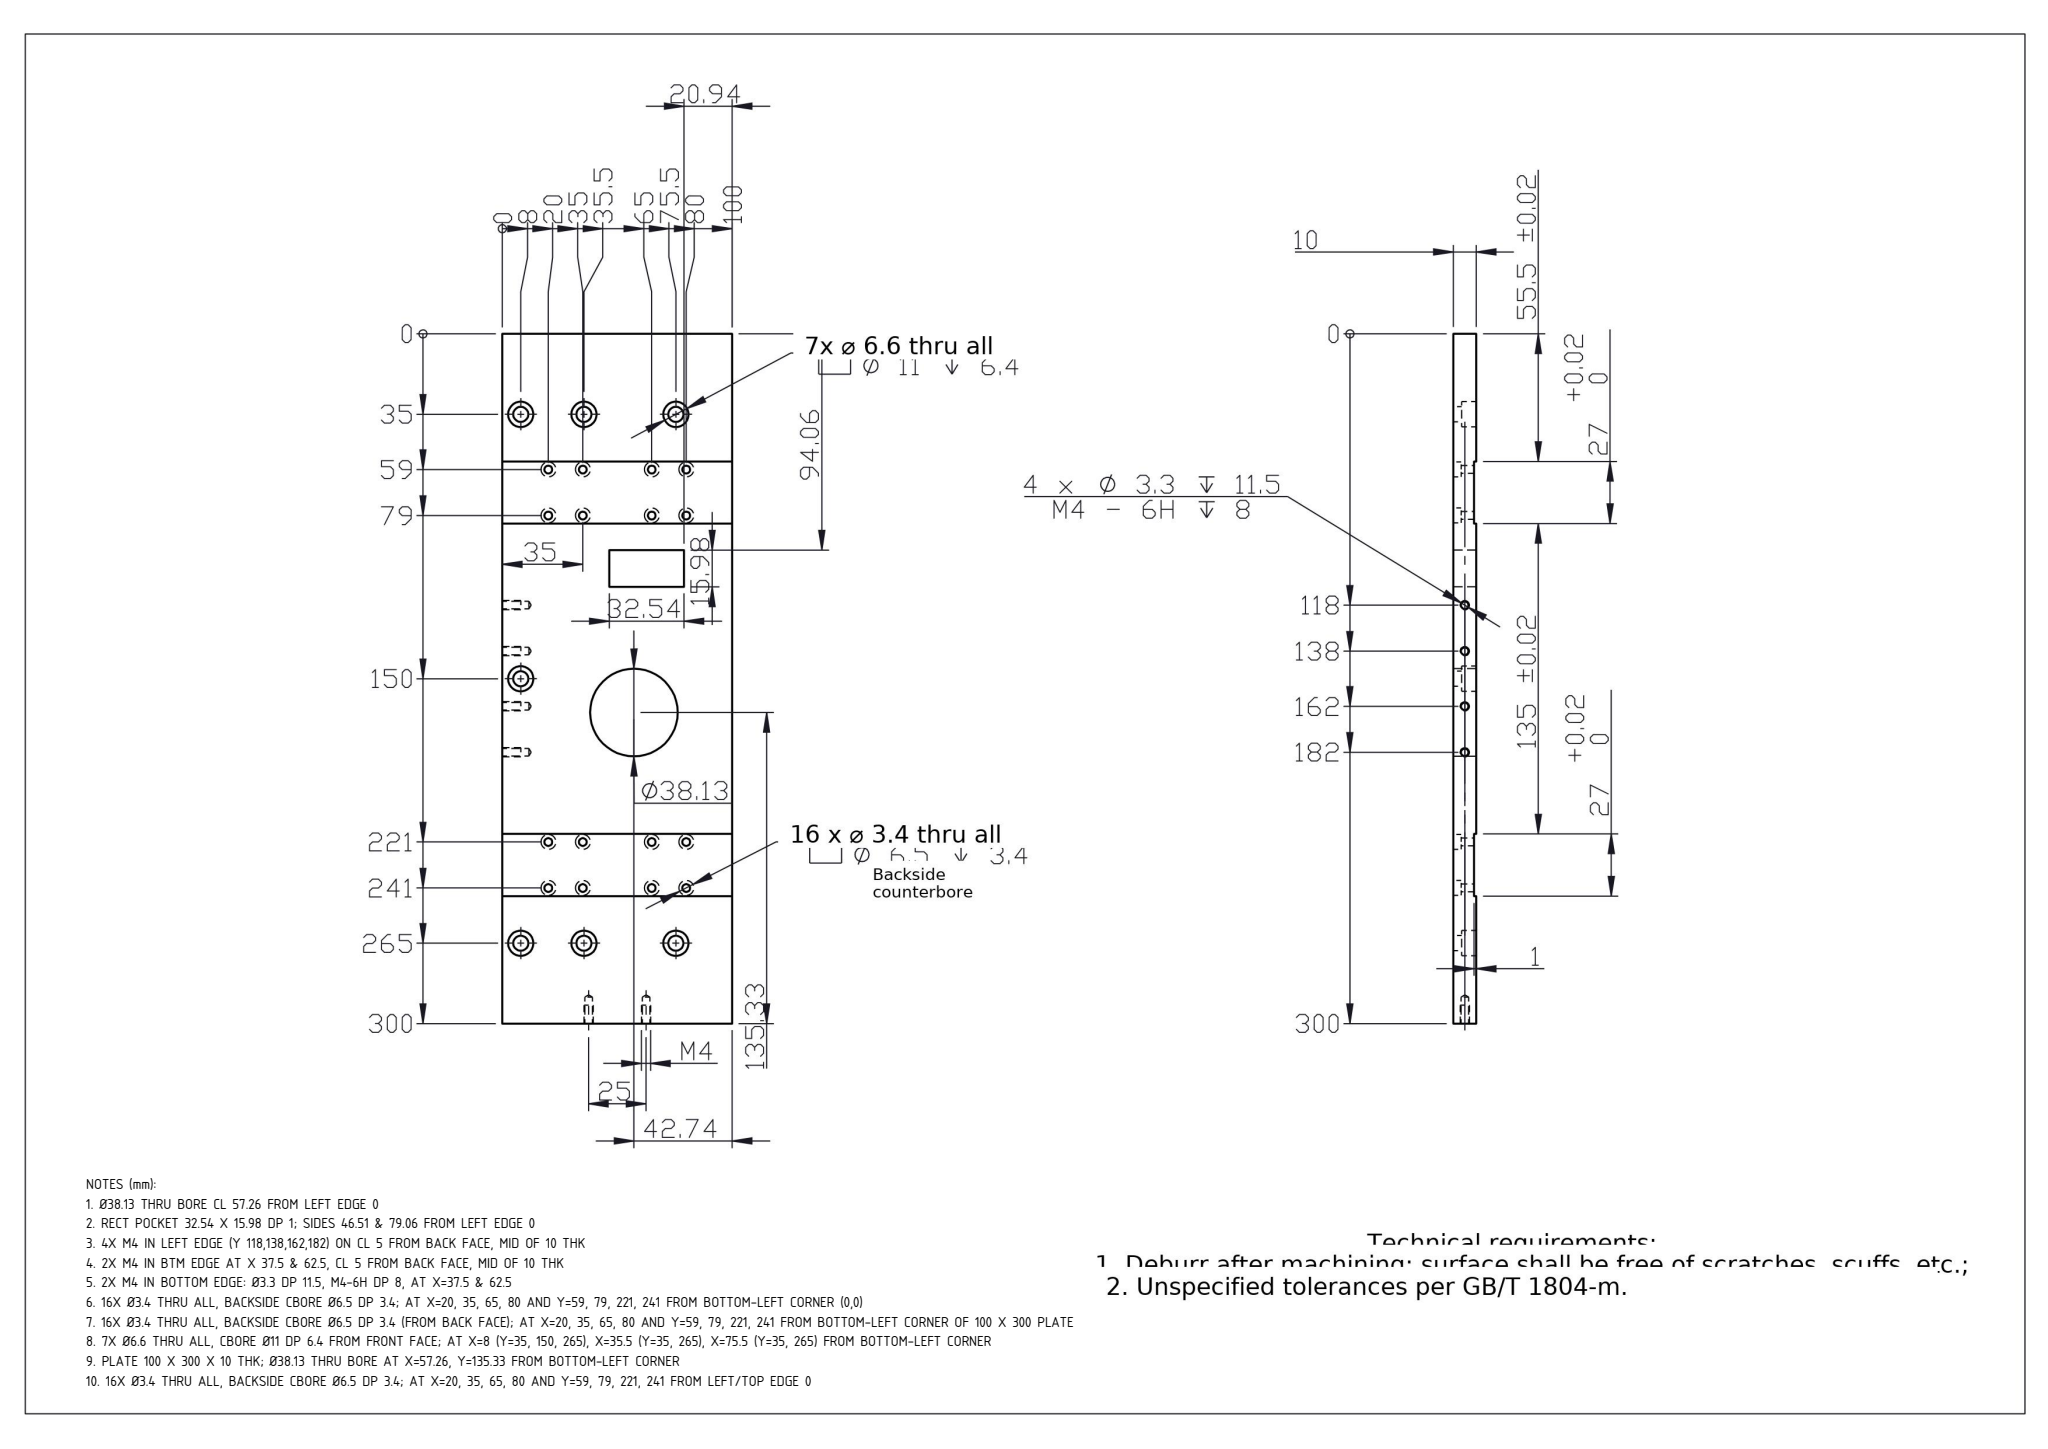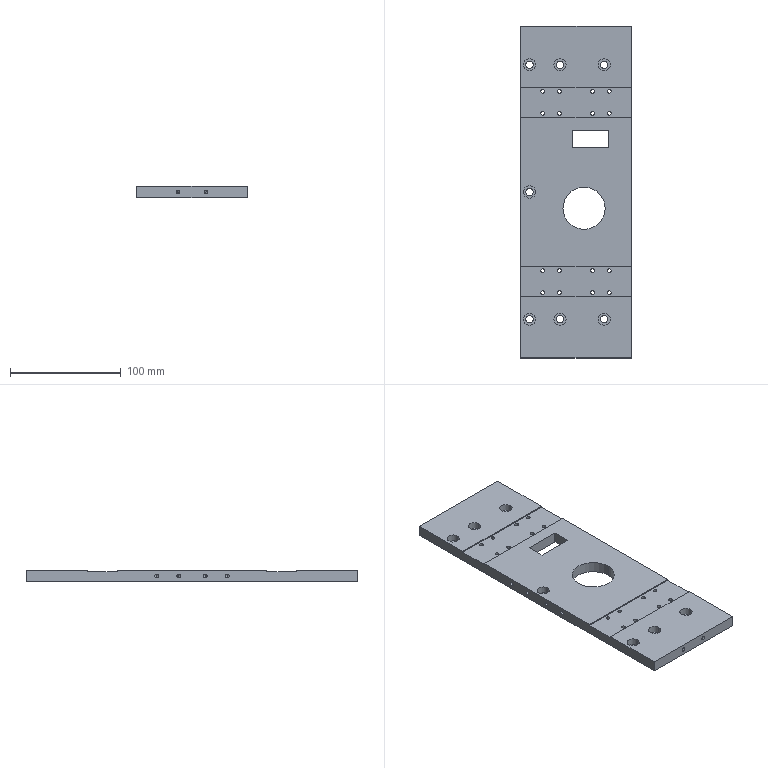Part | SolidWorks | mm | 1 solid | 159 faces | box 100 x 300 x 10 mm | volume 269636 mm3 | cylinder 106 | plane 41 | cone 12 | commonest cylinder face diameters 6.5 x32 3.4 x32 11 x14 6.6 x14 3.3 x12 38.127 x2
Drawing notes:
Ø38.13 THRU BORE CL 57.26 FROM LEFT EDGE 0 | from the solid: cyl dia38.127 axis z at (57.26,135.33), len 10 thru
RECT POCKET 32.54 X 15.98 DP 1; SIDES 46.51 & 79.06 FROM LEFT EDGE 0 | from the solid: x planes 46.51/79.06; y planes 189.95/205.94; z plane 9.0 vs top 10.0
4X M4 IN LEFT EDGE (Y 118,138,162,182) ON CL 5 FROM BACK FACE, MID OF 10 THK | from the solid: dia3.3 axis-x cyls at y=118,138,162,182, z=5.0, L=11.5; bbox z=10
2X M4 IN BTM EDGE AT X 37.5 & 62.5, CL 5 FROM BACK FACE, MID OF 10 THK | from the solid: dia3.3 axis-y cyls at x=37.5 & 62.5, z=5.0, L=11.5; bbox z=10
2X M4 IN BOTTOM EDGE: Ø3.3 DP 11.5, M4-6H DP 8, AT X=37.5 & 62.5 | from the solid: cylinders [3.3,"y",[37.5,null,5.0],11.5] and [3.3,"y",[62.5,null,5.0],11.5]; 118 deg drill point cones ref dia 3.3; matches 4X edge callout Ø3.3↧11.5 / M4-6H↧8
16X Ø3.4 THRU ALL, BACKSIDE CBORE Ø6.5 DP 3.4; AT X=20, 35, 65, 80 AND Y=59, 79, 221, 241 FROM BOTTOM-LEFT CORNER (0,0) | from the solid: cylinders dia 3.4 axis z at (20/35/65/80, 59/79/221/241) len 5.6 and dia 6.5 axis z same XY len 3.4
16X Ø3.4 THRU ALL, BACKSIDE CBORE Ø6.5 DP 3.4 (FROM BACK FACE); AT X=20, 35, 65, 80 AND Y=59, 79, 221, 241 FROM BOTTOM-LEFT CORNER OF 100 X 300 PLATE | from the solid: cylinders 3.4 dia axis z len 5.6 at (20/35/65/80, 59/79/221/241) and 6.5 dia axis z len 3.4 at same XY
7X Ø6.6 THRU ALL, CBORE Ø11 DP 6.4 FROM FRONT FACE; AT X=8 (Y=35, 150, 265), X=35.5 (Y=35, 265), X=75.5 (Y=35, 265) FROM BOTTOM-LEFT CORNER | from the solid: cylinders 6.6 dia axis z len 3.6 and 11.0 dia axis z len 6.4 at (8,35),(8,150),(8,265),(35.5,35),(35.5,265),(75.5,35),(75.5,265)
PLATE 100 X 300 X 10 THK; Ø38.13 THRU BORE AT X=57.26, Y=135.33 FROM BOTTOM-LEFT CORNER | from the solid: bbox_xyz [100,300,10]; cylinder 38.127 dia axis z len 10 at (57.26,135.33)
16X Ø3.4 THRU ALL, BACKSIDE CBORE Ø6.5 DP 3.4; AT X=20, 35, 65, 80 AND Y=59, 79, 221, 241 FROM LEFT/TOP EDGE 0 | from the solid: cylinders dia 3.4 axis z at (20/35/65/80, 59/79/221/241) len 5.6 and dia 6.5 axis z same positions len 3.4
build123d program:
from build123d import *

# Parameters (mm, degrees)
SKETCH1_W                                       = 100
SKETCH1_H                                       = 300
BOSS_EXTRUDE1_DEPTH                             = 10
SKETCH2_W                                       = 100
SKETCH2_H                                       = 27
CUT_EXTRUDE1_DEPTH                              = 1
M3_HEX_SOCKET_HEAD_CAP_SCREW_CBORE1_D           = 3.4
M3_HEX_SOCKET_HEAD_CAP_SCREW_CBORE1_CBORE_D     = 6.5
M3_HEX_SOCKET_HEAD_CAP_SCREW_CBORE1_CBORE_DEPTH = 3.4
M6_HEX_SOCKET_HEAD_CAP_SCREW_CBORE1_D           = 6.6
M6_HEX_SOCKET_HEAD_CAP_SCREW_CBORE1_CBORE_D     = 11
M6_HEX_SOCKET_HEAD_CAP_SCREW_CBORE1_CBORE_DEPTH = 6.4
M4_TAPPED_HOLE1_D                               = 3.3
M4_TAPPED_HOLE1_DEPTH                           = 11.5
M4_TAPPED_HOLE1_TIP                             = 0.9914
M6_HEX_SOCKET_HEAD_CAP_SCREW_CBORE2_D           = 6.6
M6_HEX_SOCKET_HEAD_CAP_SCREW_CBORE2_CBORE_D     = 11
M6_HEX_SOCKET_HEAD_CAP_SCREW_CBORE2_CBORE_DEPTH = 6.4
M4_TAPPED_HOLE2_D                               = 3.3
M4_TAPPED_HOLE2_DEPTH                           = 11.5
M4_TAPPED_HOLE2_TIP                             = 0.9914
SKETCH14_R                                      = 19.063
SKETCH14_W                                      = 32.545
SKETCH14_H                                      = 15.982
CUT_EXTRUDE2_DEPTH                              = 59


with BuildPart() as part:
    # Sketch1 → Boss-Extrude1 (new body)
    with BuildSketch(Plane.XY):
        with Locations((50, -150)):
            Rectangle(SKETCH1_W, SKETCH1_H)
    extrude(amount=BOSS_EXTRUDE1_DEPTH)

    # Sketch2 → Cut-Extrude1 (cut)
    with BuildSketch(Plane.XY.offset(10)):
        with Locations((50, -69)):
            Rectangle(SKETCH2_W, SKETCH2_H)
        with Locations((50, -231)):
            Rectangle(SKETCH2_W, SKETCH2_H)
    extrude(amount=-CUT_EXTRUDE1_DEPTH, mode=Mode.SUBTRACT)

    # M3 Hex Socket Head Cap Screw CBORE1 (through all)
    with Locations(Plane(origin=(-13.017, -41.166, 0), x_dir=(1, 0, 0), z_dir=(0, 0, -1))):
        with Locations((33.017, 17.834), (48.017, 17.834), (33.017, 37.834), (48.017, 37.834), (78.017, 17.834), (93.017, 17.834), (93.017, 37.834), (78.017, 37.834), (33.017, 179.834), (48.017, 179.834), (48.017, 199.834), (33.017, 199.834), (78.017, 179.834), (93.017, 179.834), (93.017, 199.834), (78.017, 199.834)):
            CounterBoreHole(M3_HEX_SOCKET_HEAD_CAP_SCREW_CBORE1_D / 2, M3_HEX_SOCKET_HEAD_CAP_SCREW_CBORE1_CBORE_D / 2, M3_HEX_SOCKET_HEAD_CAP_SCREW_CBORE1_CBORE_DEPTH)

    # M6 Hex Socket Head Cap Screw CBORE1 (through all)
    with Locations(Plane.XY.offset(10)):
        with Locations((8, -35), (8, -150), (8, -265)):
            CounterBoreHole(M6_HEX_SOCKET_HEAD_CAP_SCREW_CBORE1_D / 2, M6_HEX_SOCKET_HEAD_CAP_SCREW_CBORE1_CBORE_D / 2, M6_HEX_SOCKET_HEAD_CAP_SCREW_CBORE1_CBORE_DEPTH)

    # M4 Tapped Hole1
    with Locations(Plane.ZY):
        with Locations((5, -118), (5, -138), (5, -162), (5, -182)):
            Hole(M4_TAPPED_HOLE1_D / 2, depth=M4_TAPPED_HOLE1_DEPTH)
            with Locations((0, 0, -(M4_TAPPED_HOLE1_DEPTH + M4_TAPPED_HOLE1_TIP / 2))):  # 118° drill point
                Cone(0, M4_TAPPED_HOLE1_D / 2, M4_TAPPED_HOLE1_TIP, mode=Mode.SUBTRACT)

    # M6 Hex Socket Head Cap Screw CBORE2 (through all)
    with Locations(Plane.XY.offset(10)):
        with Locations((35.5, -265), (75.5, -265), (35.5, -35), (75.5, -35)):
            CounterBoreHole(M6_HEX_SOCKET_HEAD_CAP_SCREW_CBORE2_D / 2, M6_HEX_SOCKET_HEAD_CAP_SCREW_CBORE2_CBORE_D / 2, M6_HEX_SOCKET_HEAD_CAP_SCREW_CBORE2_CBORE_DEPTH)

    # M4 Tapped Hole2
    with Locations(Plane(origin=(0, -300, 0), x_dir=(-1, 0, 0), z_dir=(0, -1, 0))):
        with Locations((-37.5, -5), (-62.5, -5)):
            Hole(M4_TAPPED_HOLE2_D / 2, depth=M4_TAPPED_HOLE2_DEPTH)
            with Locations((0, 0, -(M4_TAPPED_HOLE2_DEPTH + M4_TAPPED_HOLE2_TIP / 2))):  # 118° drill point
                Cone(0, M4_TAPPED_HOLE2_D / 2, M4_TAPPED_HOLE2_TIP, mode=Mode.SUBTRACT)

    # Sketch14 → Cut-Extrude2 (cut)
    with BuildSketch(Plane.XY.offset(10)):
        with Locations((57.264, -164.674)):
            Circle(SKETCH14_R)
        with Locations((62.785, -102.055)):
            Rectangle(SKETCH14_W, SKETCH14_H)
    extrude(amount=-CUT_EXTRUDE2_DEPTH, mode=Mode.SUBTRACT)


solid = part.part